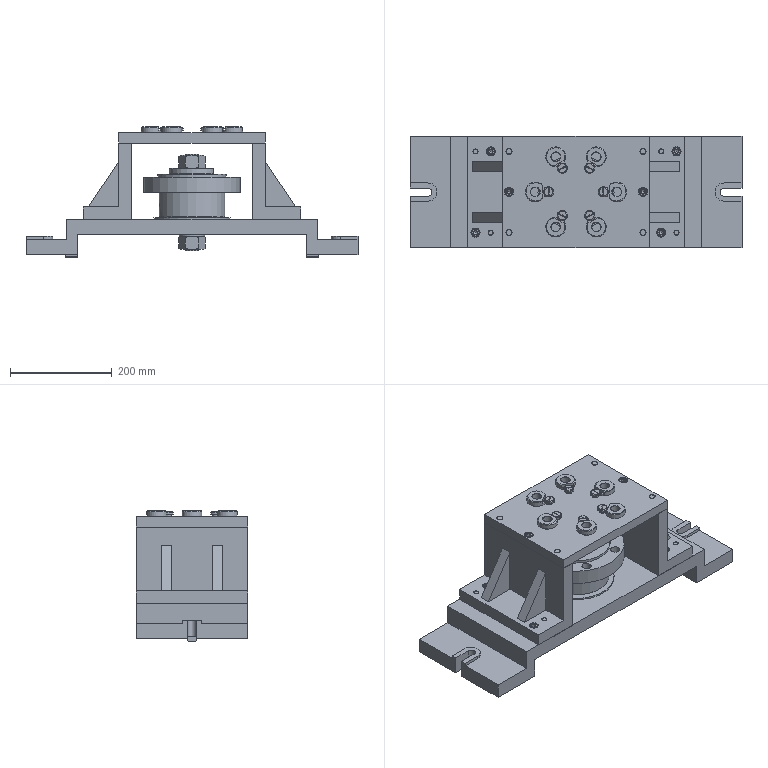Assembly | NX | mm | 40 component files | 40 solids | 696 faces | box 654 x 220 x 257 mm | volume 10168790 mm3 | plane 350 | cone 179 | cylinder 151 | torus 16 | commonest cylinder face diameters 10 x20 18 x18 12 x18 26 x12 8 x12 6 x8 16 x8 11 x8
Bill of materials:
unnamed part 1 | 6 |  | Axisymmetric headed pin/screw-like part: a round head with a chamfered top edge and a straight slot across it, a cylindrical shoulder under the head, a short neck of smaller diameter, then a plain cylindrical shank.
GB-T70.1-2000,M10x20 | 2 |  | Hexagon Socket Head Cap Screw, GB-T 70.1-2000,M10x20
GB-T70.1-2000,M10x25 | 4 |  | Hexagon Socket Head Cap Screw, GB-T 70.1-2000,M10x25
GB-T119.1-2000,10x40 | 4 |  | Parallel Pin, GB-T 119.1-2000,10x40
unnamed part 2 | 2 |  | Rectangular block with chamfered long edges and one round through hole in the middle of the top face.
unnamed part 3 | 6 |  | Flanged sleeve/bushing: a cylindrical body with a larger round flange at one end, a through bore, chamfered edges, and a local notch or flat-bottomed cutout on the edge of the flange.
GB-T70.1-2000,M6x10 | 2 |  | Hexagon Socket Head Cap Screw, GB-T 70.1-2000,M6x10
GB-T95-2002,M27 | 1 |  | Plain Washer, GB-T 95-2002,M27
unnamed part 4 | 1 |  | Flanged hub: a round flange with six through holes spaced evenly on a bolt circle, a raised annular boss on the top face, a central through bore, and a cylindrical spigot/body below the flange.
GB-T119.1-2000,12x40 | 4 |  | Parallel Pin, GB-T 119.1-2000,12x40
GB-T6170_F-2000,M30x3.5 | 2 |  | Hexagonal nut-like body with a central round through bore, double-chamfered corners (curved chamfer arcs on the flats at both faces), and chamfered or countersunk bore entries.
unnamed part 5 | 1 |  | Flat circular disk with an open slot running from the outer edge to past the center and ending in a semicircle (C- or U-shaped washer outline), with lightly chamfered edges.
unnamed part 6 | 1 |  | Flat rectangular plate with a symmetric pattern of holes: six small through holes near the two short edges, six larger through holes in a circular arrangement, and six small blind holes inside that ring.
unnamed part 7 | 1 |  | Solid stepped cylindrical pin: a larger-diameter central cylinder with smaller coaxial cylindrical ends extending from both faces.
unnamed part 8 | 1 |  | Long plate with a stepped (hat-like) profile: a raised central section and lower end tabs, each tab with an open-ended U-slot. In the center is a round through hole with a shallow circular raised pad, and there are four pairs of small holes.
unnamed part 9 | 2 |  | L-shaped bracket: a tall upright wall on a base flange, with sloped gusset/support geometry between them. It has holes in the top edge of the wall and in the base, plus rectangular pockets on the underside.
Mates:
1. fix | fixture_body 1 component
2. concentric | locating_pin 1 edge | fixture_body 1 edge
3. concentric | cylinder_head_body 1 edge | fixture_body 1 edge
4. concentric | quick_change_washer 1 edge | cylinder_head_body 1 edge
5. concentric | GB-T6170_F-2000_M30x3_5 2 edge | quick_change_washer 1 edge
6. concentric | GB-T95-2002_M27 1 edge | fixture_body 1 edge
7. concentric | GB-T6170_F-2000_M30x3_5 1 edge | GB-T95-2002_M27 1 edge
8. touch align | angle_iron 2 face | fixture_body 1 face
9. distance | angle_iron 2 face | locating_pin 1 face
10. touch align | angle_iron 2 face | fixture_body 1 face
11. bond | cylinder_head_body 1 component | assembly component
12. bond | angle_iron 2 component | assembly component
13. bond | angle_iron 1 component | assembly component
14. circular | assembly datumaxis | assembly cartesiancoordinatesystem | assembly cartesiancoordinatesystem
15. touch align | drill_template 1 face | angle_iron 1 face
16. touch align | drill_template 1 face | angle_iron 2 face
17. touch align | drill_template 1 face | angle_iron 2 face
18. concentric | drill_bush 6 edge | drill_template 1 edge
19. concentric | drill_bush_screw 6 edge | drill_template 1 arc
20. bond | cylinder_head_body 1 component | assembly component
21. bond | drill_bush 6 component | assembly component
22. bond | drill_bush_screw 6 component | assembly component
23. bond | drill_bush 5 component | assembly component
24. bond | drill_bush_screw 5 component | assembly component
25. circular | assembly datumaxis | assembly cartesiancoordinatesystem | assembly cartesiancoordinatesystem | assembly cartesiancoordinatesystem | assembly cartesiancoordinatesystem | assembly cartesiancoordinatesystem | assembly cartesiancoordinatesystem
26. circular | assembly datumaxis | assembly cartesiancoordinatesystem | assembly cartesiancoordinatesystem | assembly cartesiancoordinatesystem | assembly cartesiancoordinatesystem | assembly cartesiancoordinatesystem | assembly cartesiancoordinatesystem
27. bond | drill_bush 4 component | assembly component
28. bond | drill_bush_screw 4 component | assembly component
29. bond | drill_bush 3 component | assembly component
30. bond | drill_bush_screw 3 component | assembly component
31. bond | drill_bush 2 component | assembly component
32. bond | drill_bush_screw 2 component | assembly component
33. bond | drill_bush 1 component | assembly component
34. bond | drill_bush_screw 1 component | assembly component
35. concentric | GB-T119_1-2000_10x40 4 edge | angle_iron 2 edge
36. concentric | GB-T70_1-2000_M10x25 3 edge | angle_iron 2 edge
37. concentric | GB-T119_1-2000_10x40 2 edge | angle_iron 1 edge
38. concentric | GB-T70_1-2000_M10x25 1 edge | angle_iron 1 edge
39. touch align | locating_key 2 face | fixture_body 1 face
40. touch align | locating_key 2 face | fixture_body 1 face
41. touch align | locating_key 2 face | fixture_body 1 face
42. bond | fixture_body 1 component | assembly component
43. bond | locating_key 2 component | assembly component
44. bond | locating_key 1 component | assembly component
45. linear | assembly datumaxis | assembly cartesiancoordinatesystem | assembly cartesiancoordinatesystem
46. fix | GB-T6170_F-2000_M30x3_5 2 component
47. fix | cylinder_head_body 1 component